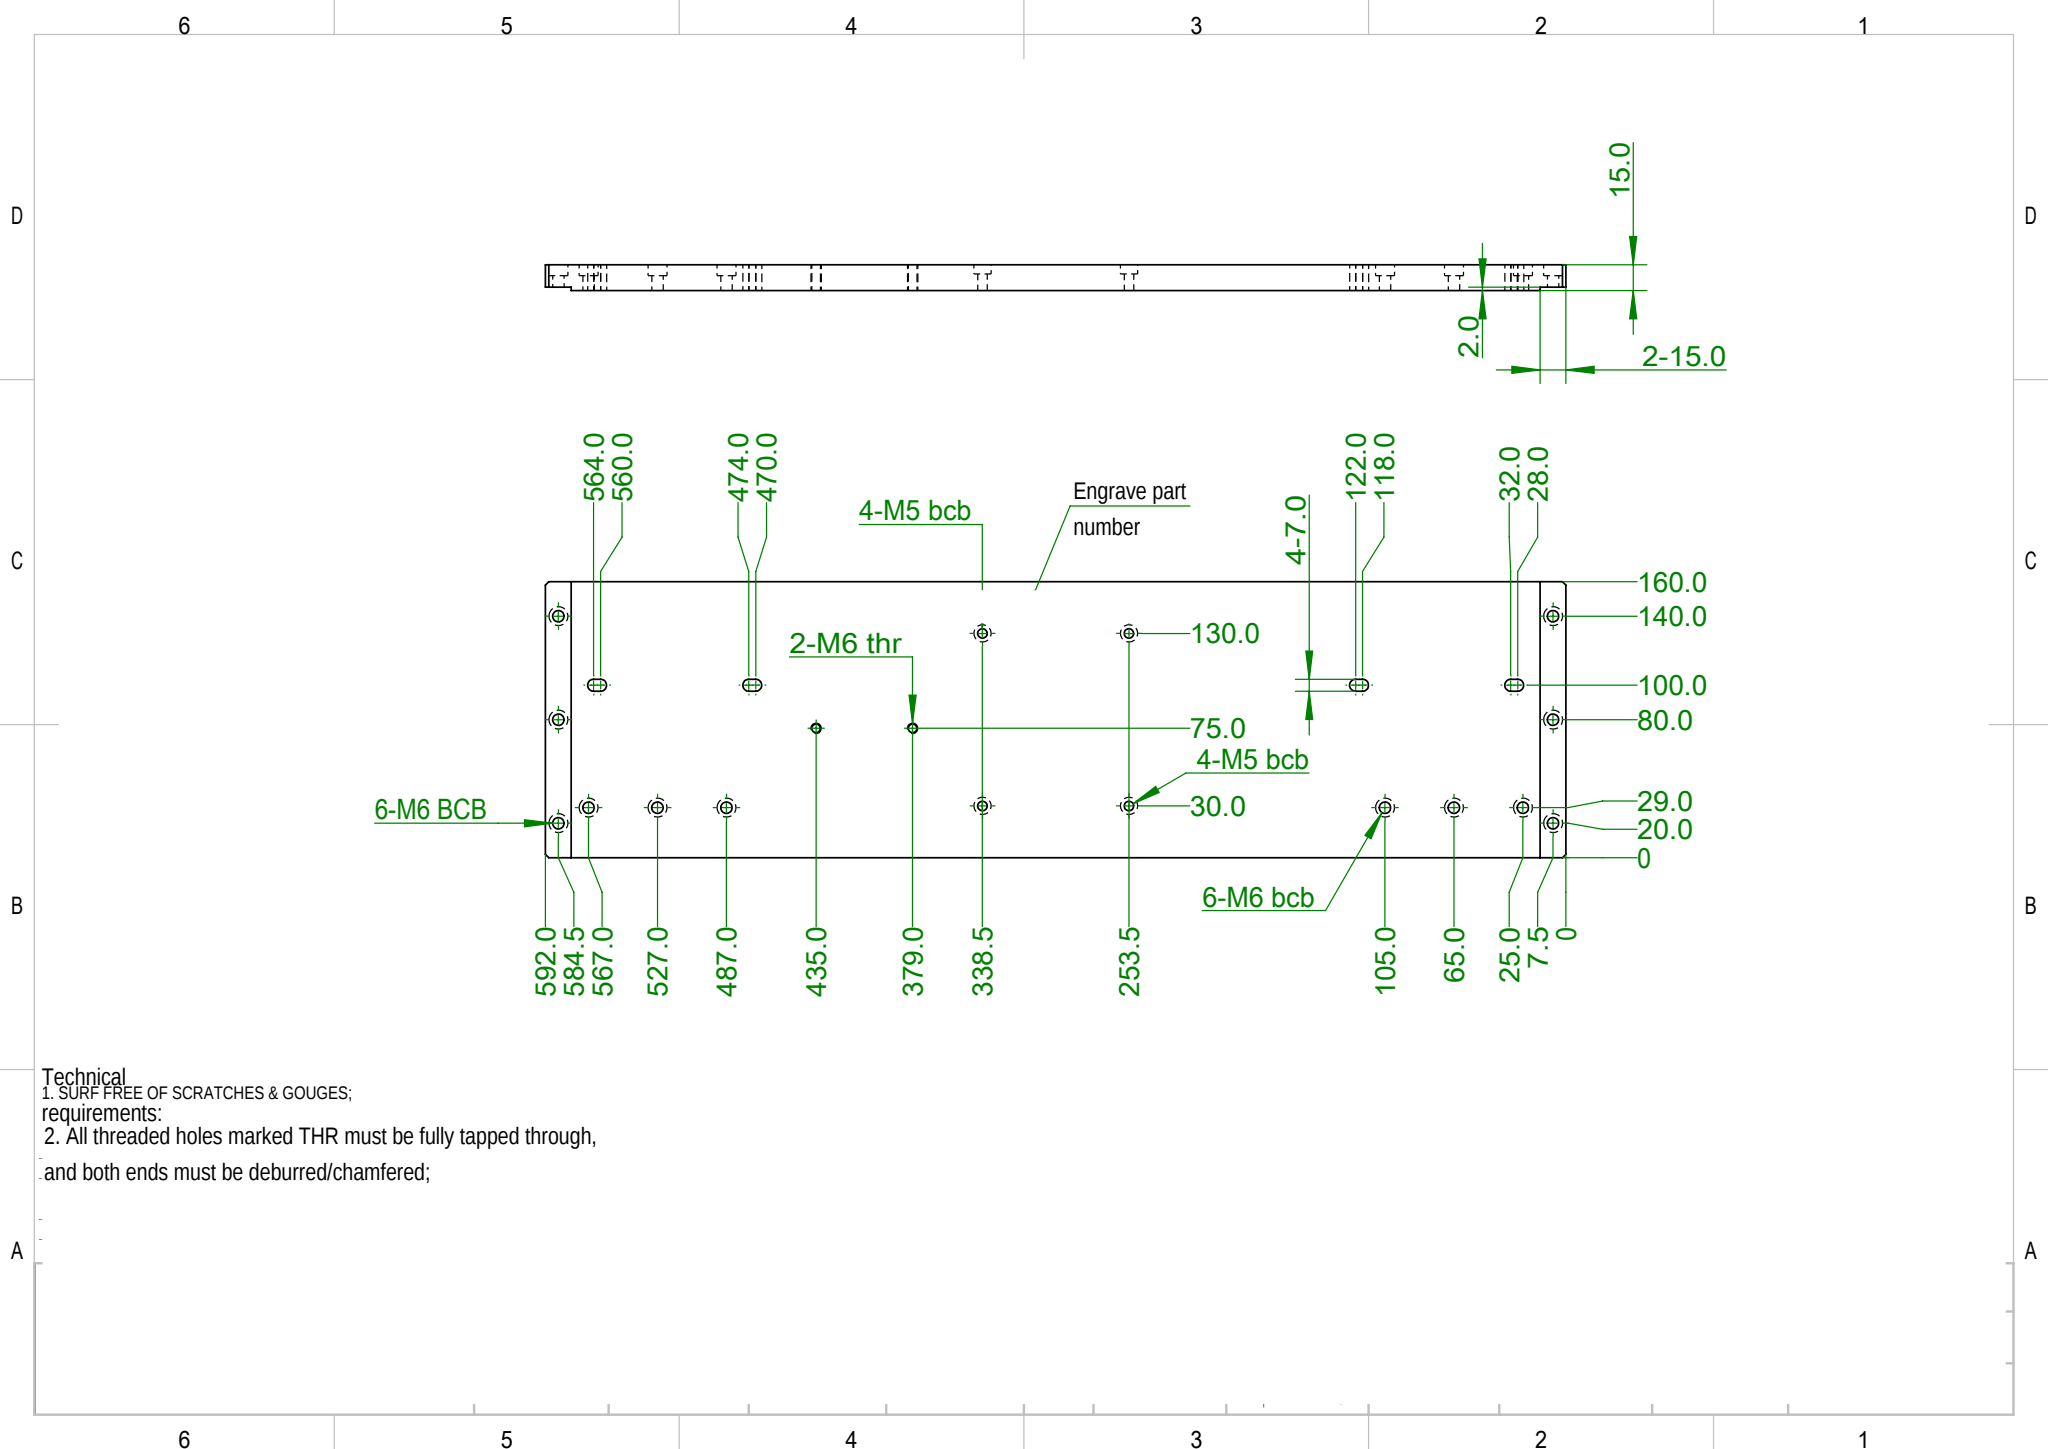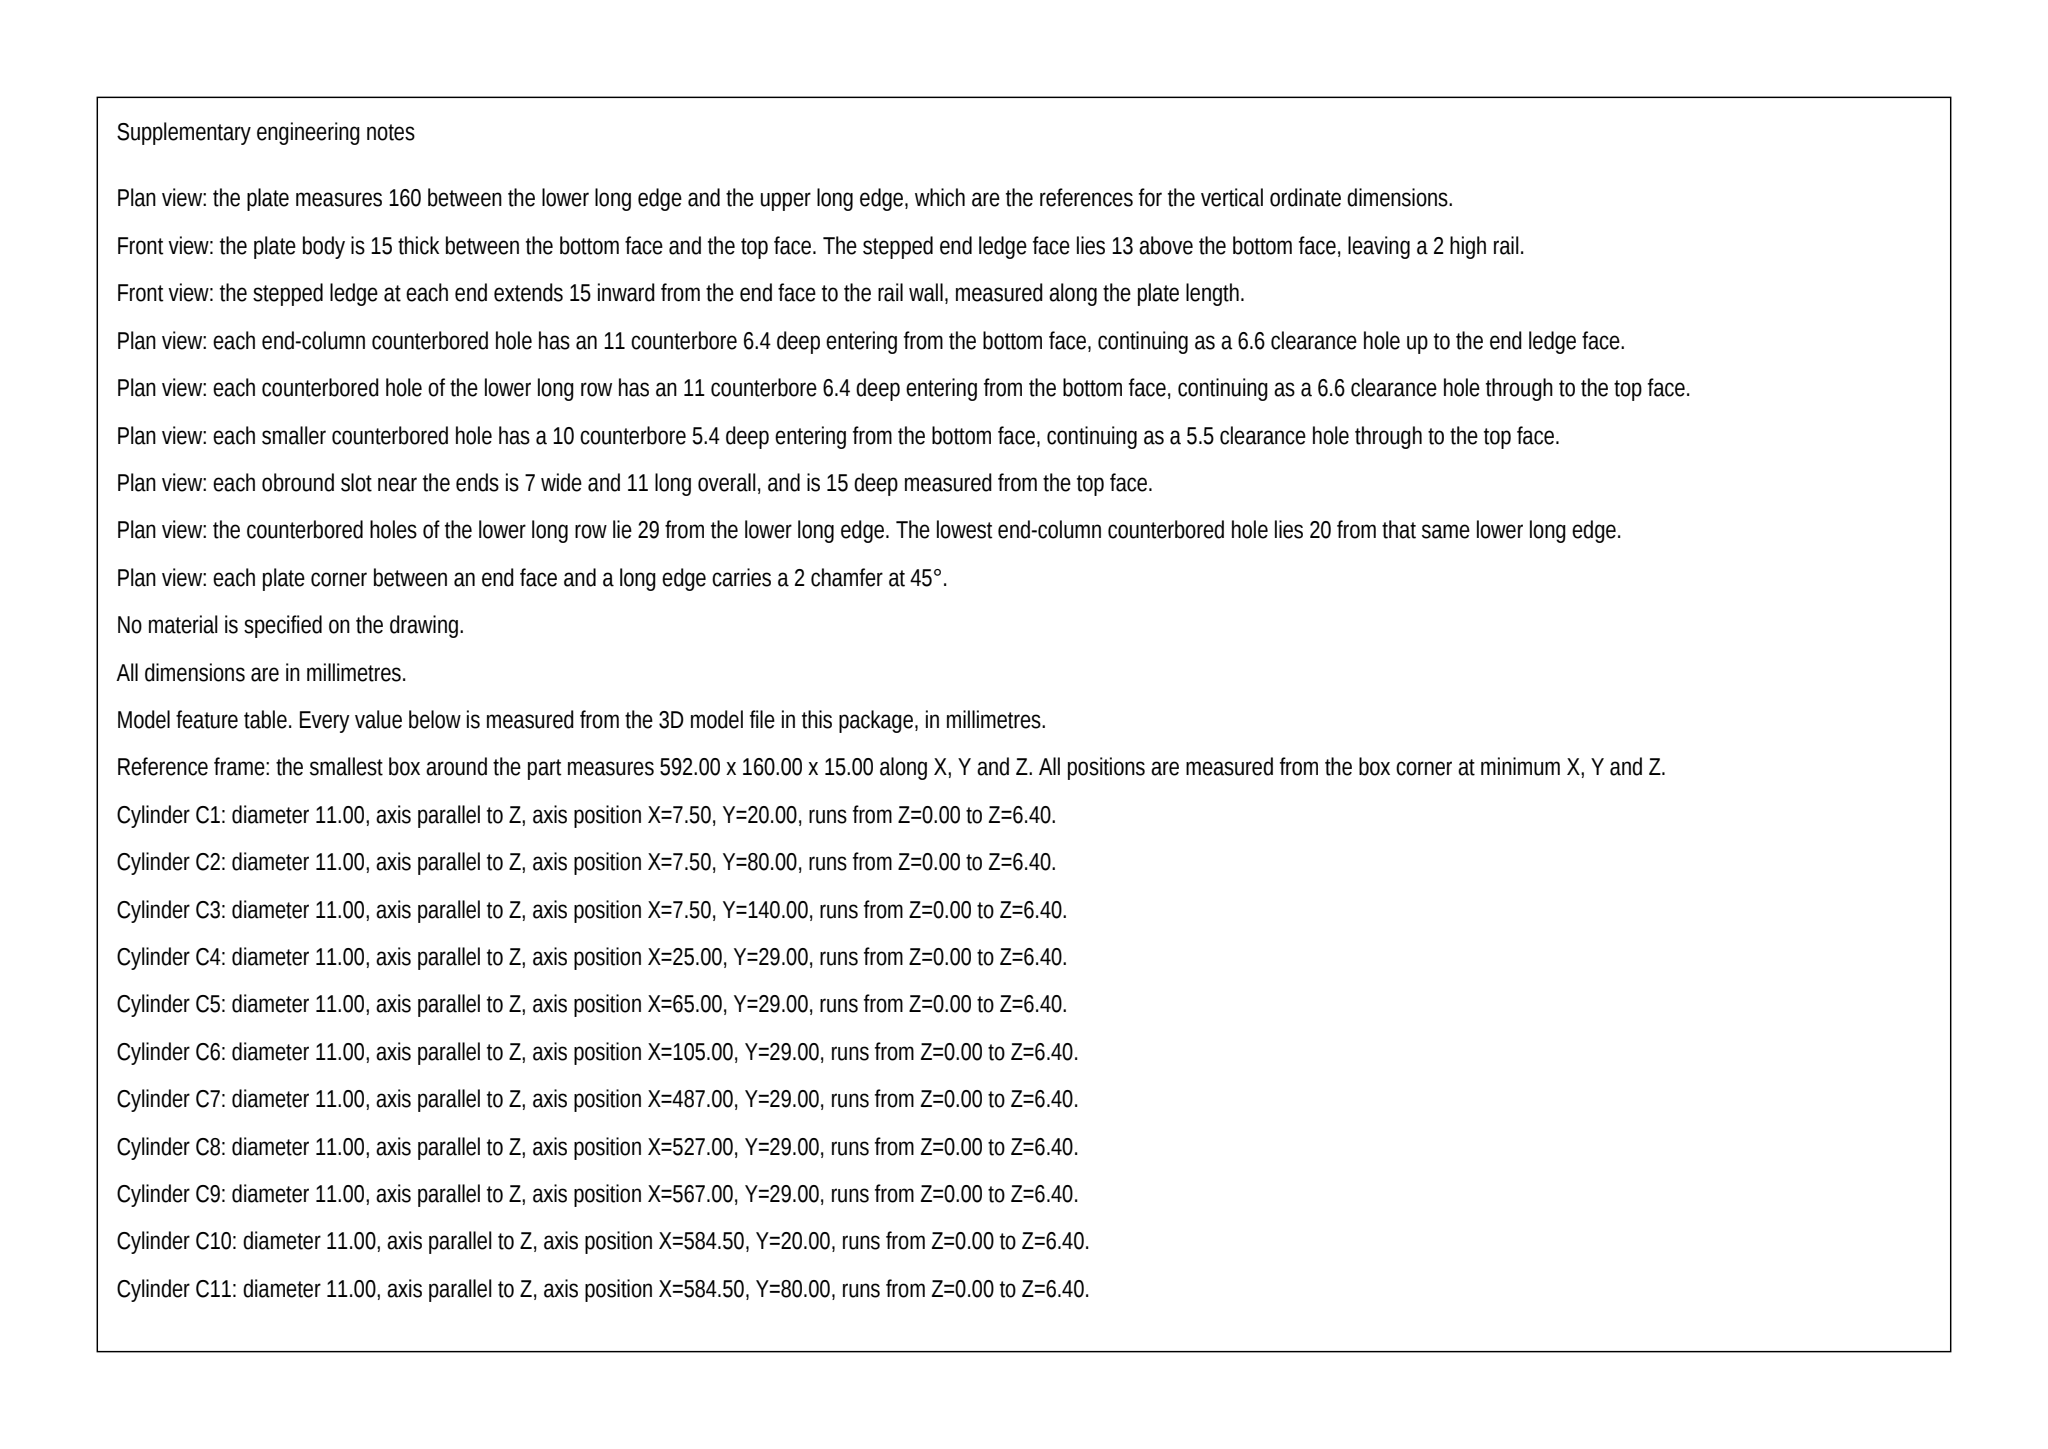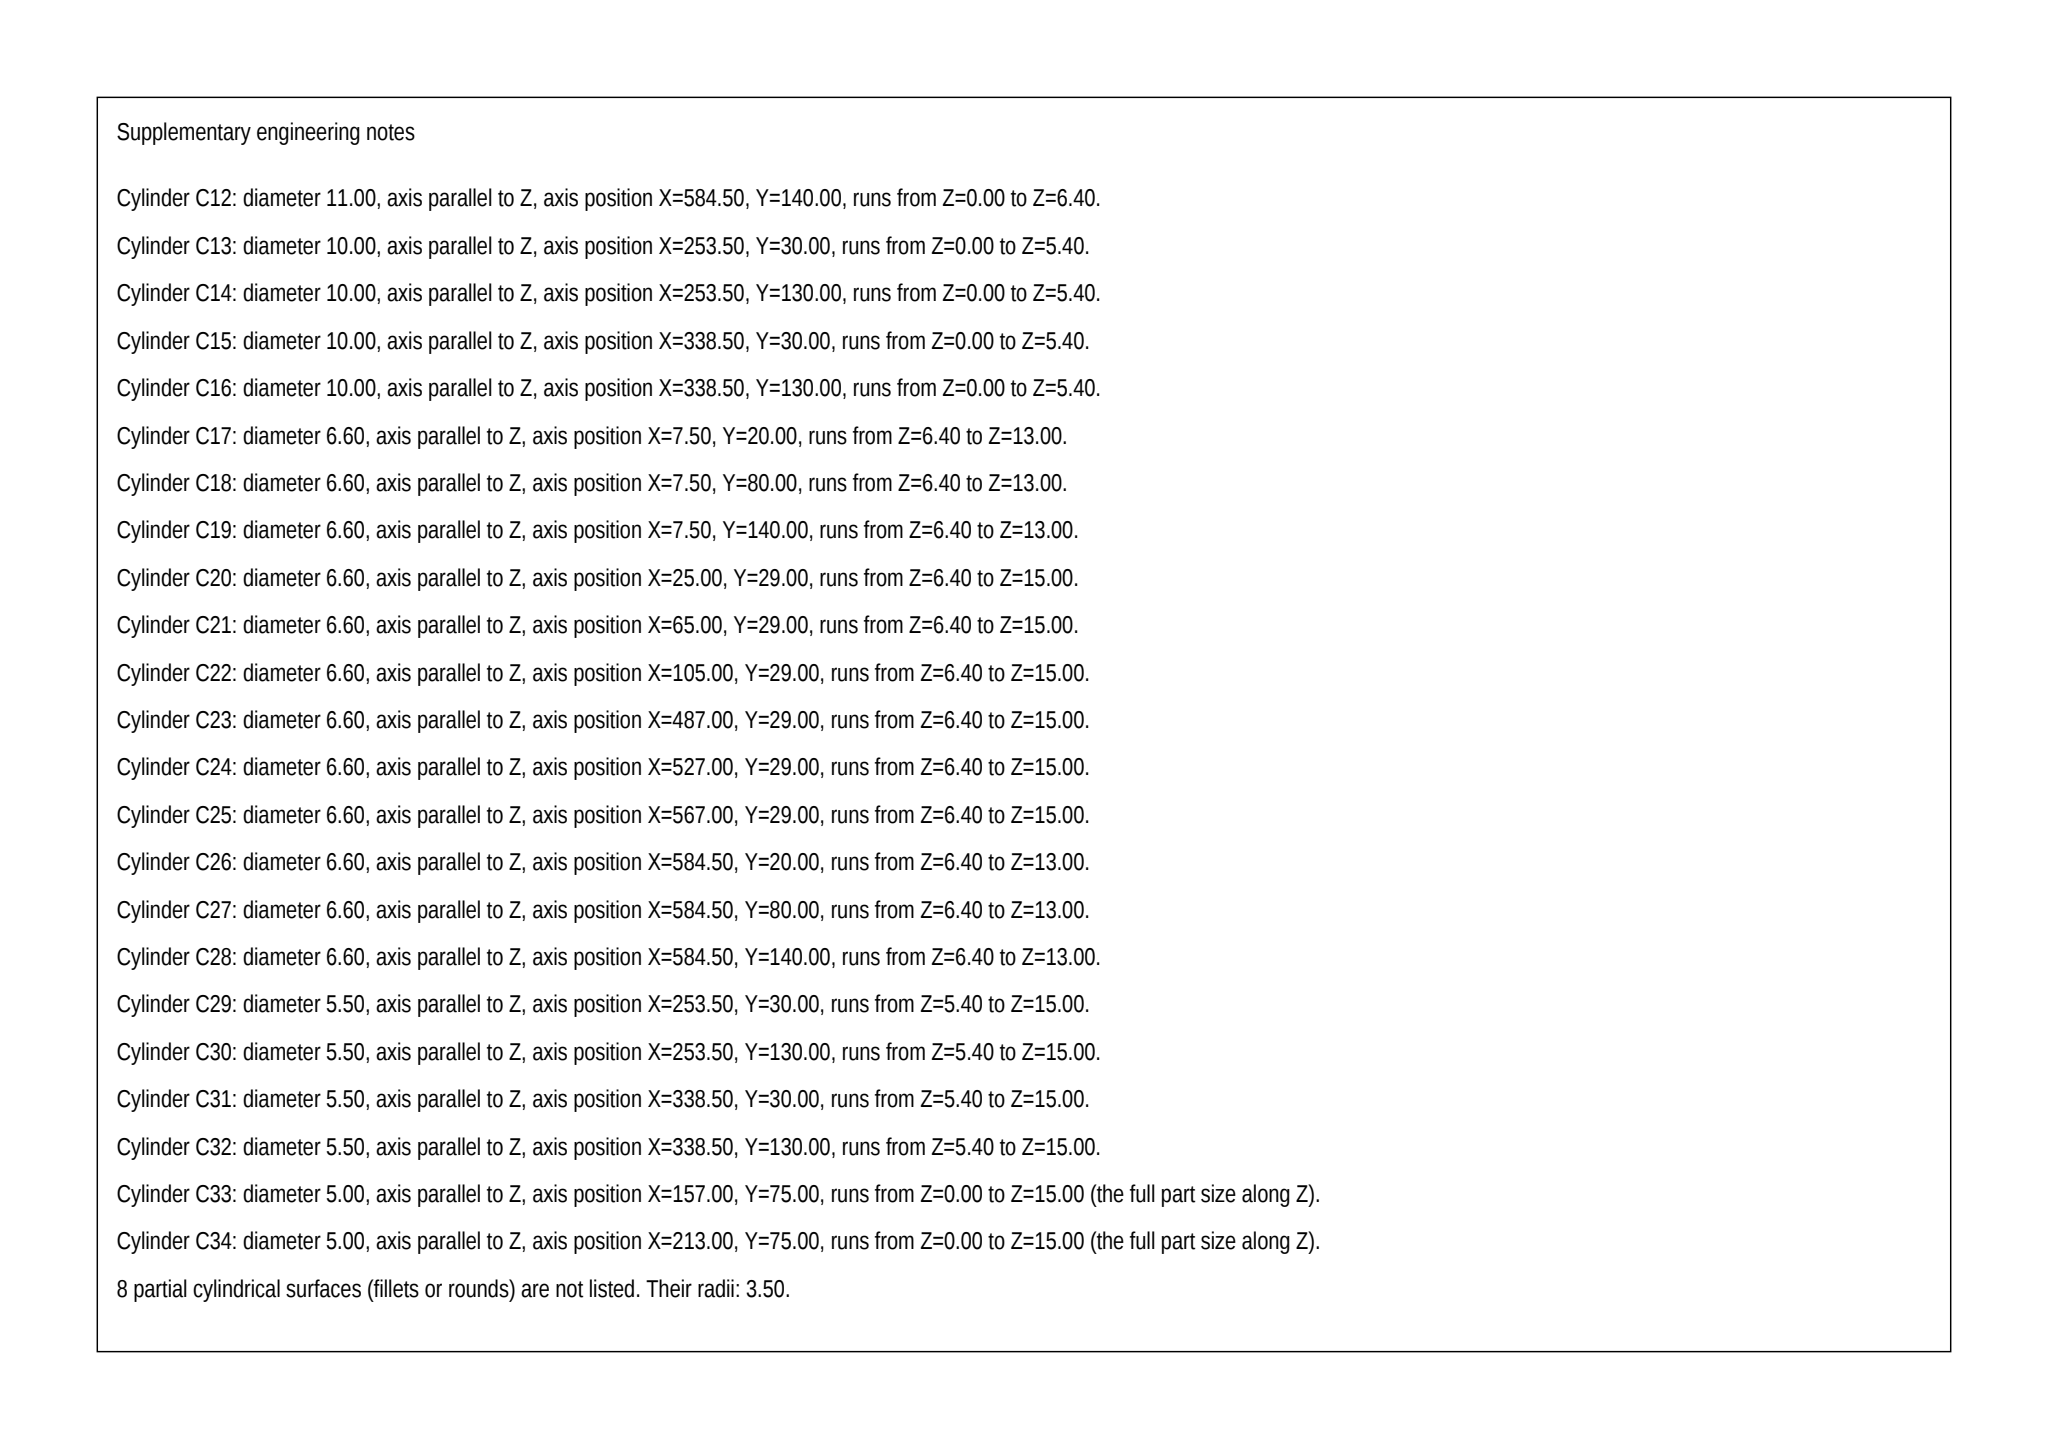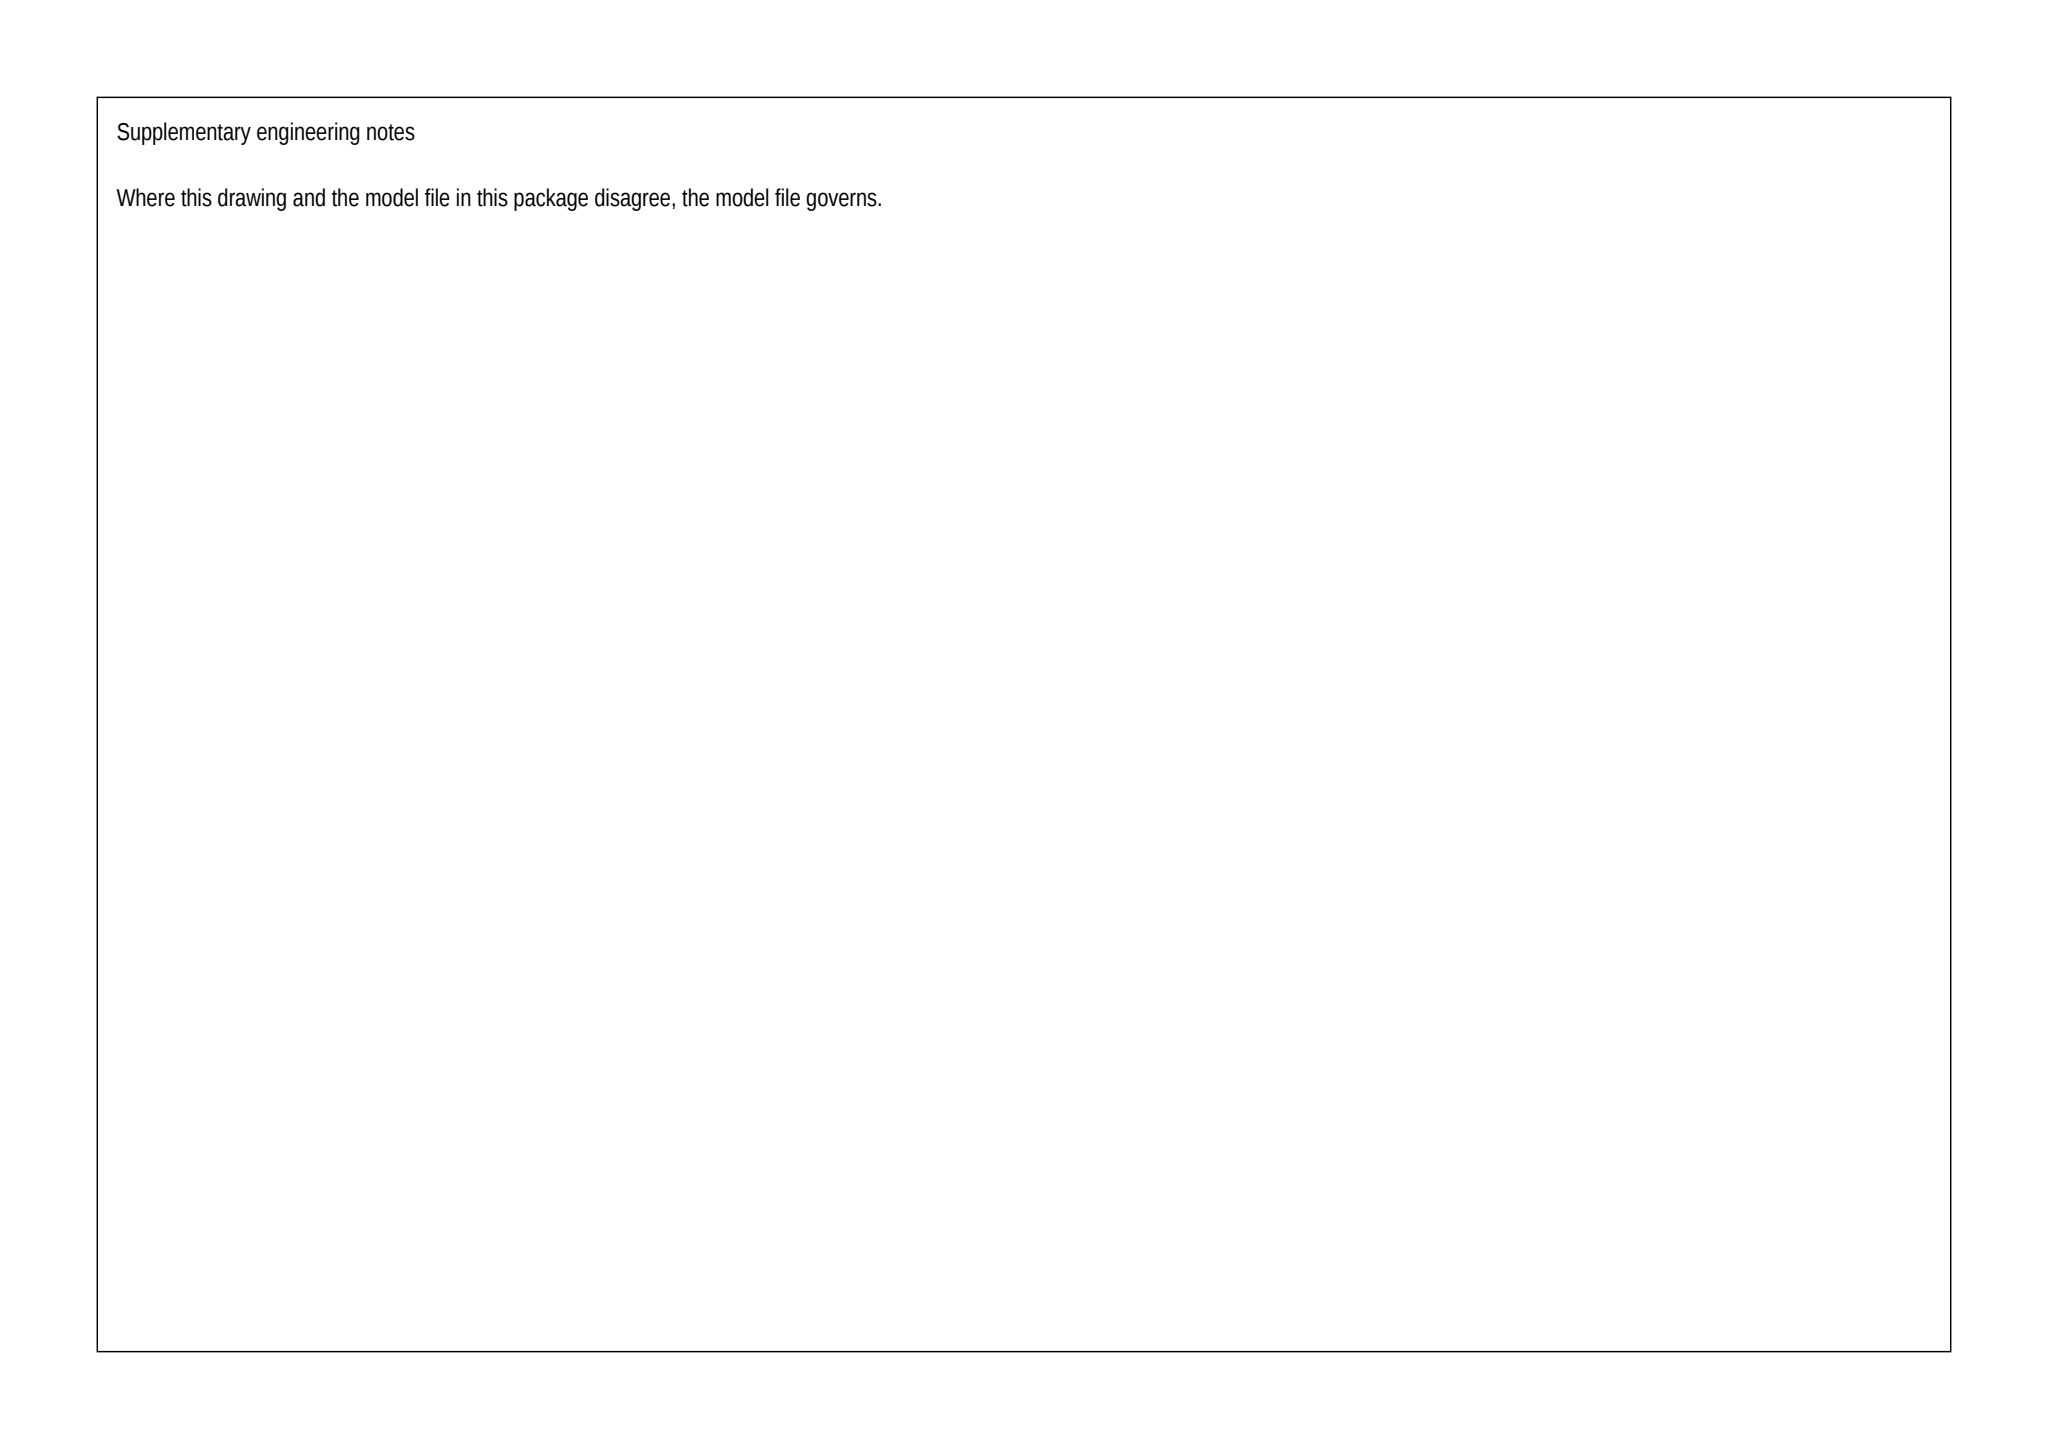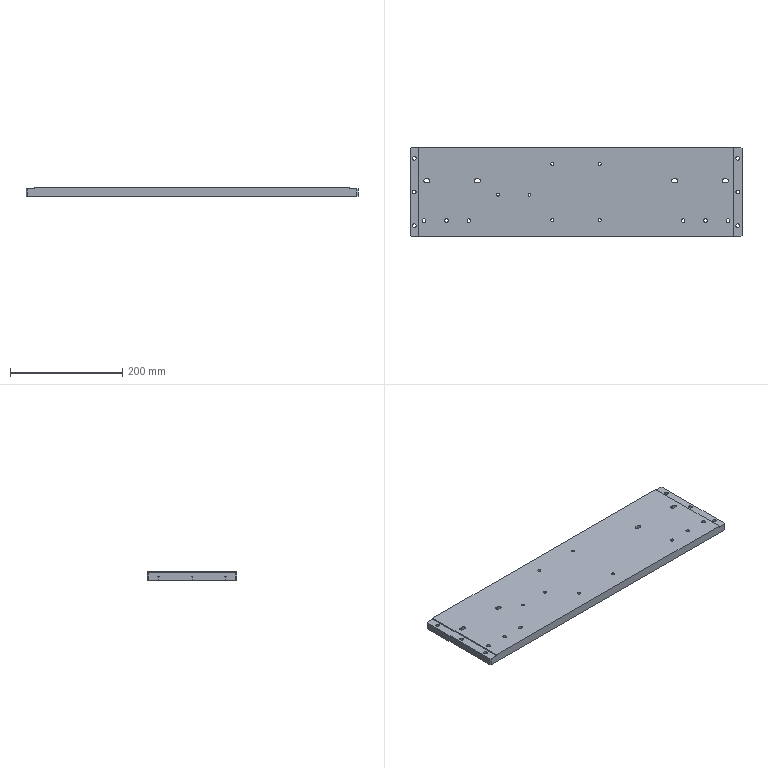Part | SolidWorks | mm | 1 solid | 118 faces | box 592 x 160 x 15 mm | volume 1393490 mm3 | cylinder 80 | plane 38 | commonest cylinder face diameters 11 x24 6.6 x24 7 x12 10 x8 5.5 x8 5 x4
Drawing notes:
12X Ø6.6 THRU, C'BORE Ø11.0 DEEP 6.4 from top face; located from bbox min corner at (X7.5,Y20), (X7.5,Y80), (X7.5,Y140), (X584.5,Y20), (X584.5,Y80), (X584.5,Y140), and (X25,Y29), (X65,Y29), (X105,Y29), (X487,Y29), (X527,Y29), (X567,Y29). | from the solid: cylinders dia 6.6 (12 locations, len 6.6/8.6) with coaxial dia 11.0 depth 6.4 at same XY
4X Ø5.5 THRU, C'BORE Ø10.0 DEEP 5.4 from top face; located from bbox min corner at (X253.5,Y30), (X253.5,Y130), (X338.5,Y30), (X338.5,Y130). | from the solid: cylinders dia 5.5 len 9.6 at (253.5/338.5, 30/130) with coaxial dia 10.0 depth 5.4
4X Ø7.0 THRU slots, full 15.0 plate thickness, slot centerline Y=100.0 from bbox min corner; end-radius centers at X=28.0 & 32.0, X=118.0 & 122.0, X=470.0 & 474.0, X=560.0 & 564.0. | from the solid: cylinders dia 7.0 axis z len 15.0 at y=100.0, x=28/32, 118/122, 470/474, 560/564
2X M6 TAPPED THRU (tap drill Ø5.0 through 15.0 thickness), located from bbox min corner at (X157.0,Y75.0) and (X213.0,Y75.0). | from the solid: cylinders dia 5.0 axis z len 15.0 at (157.0,75.0) and (213.0,75.0)
All dimensions are in millimetres; overall part size 592.0 x 160.0 x 15.0. | from the solid: bbox_xyz [592.0,160.0,15.0] with units mm
SLOT: 4X Ø7.0 THRU slots, full 15.0 plate thickness; slot centerline Y=100.0 from bbox min corner; end-radius centers at X=118.0 and X=122.0 from bbox min corner (X0,Y0 = bbox min corner). | from the solid: cylinders dia 7.0, axis z, pos (118.0,100.0) and (122.0,100.0), length 15.0 = full 15.0 plate thickness; bbox_xyz 592.0 x 160.0 x 15.0
build123d program:
from build123d import *

# Parameters (mm, degrees)
SKETCH1_W                                       = 590
SKETCH1_H                                       = 160
BOSS_EXTRUDE1_DEPTH                             = 15
SKETCH2_W                                       = 14
SKETCH2_H                                       = 160
CUT_EXTRUDE1_DEPTH                              = 2
M5_HEX_SOCKET_HEAD_CAP_SCREW_CBORE1_D           = 5.5
M5_HEX_SOCKET_HEAD_CAP_SCREW_CBORE1_CBORE_D     = 10
M5_HEX_SOCKET_HEAD_CAP_SCREW_CBORE1_CBORE_DEPTH = 5.4
MOVE_FACE1_BY                                   = 1
MOVE_FACE2_BY                                   = 1
CUT_EXTRUDE3_DEPTH                              = 111
M6_HEX_SOCKET_HEAD_CAP_SCREW_CBORE1_D           = 6.6
M6_HEX_SOCKET_HEAD_CAP_SCREW_CBORE1_CBORE_D     = 11
M6_HEX_SOCKET_HEAD_CAP_SCREW_CBORE1_CBORE_DEPTH = 6.4
M6_HEX_SOCKET_HEAD_CAP_SCREW_CBORE2_D           = 6.6
M6_HEX_SOCKET_HEAD_CAP_SCREW_CBORE2_CBORE_D     = 11
M6_HEX_SOCKET_HEAD_CAP_SCREW_CBORE2_CBORE_DEPTH = 6.4
M6_TAPPED_HOLE1_D                               = 5
CHAMFER1_SIZE                                   = 2


with BuildPart() as part:
    # Sketch1 → Boss-Extrude1 (new body)
    with BuildSketch(Plane.XY):
        Rectangle(SKETCH1_W, SKETCH1_H)
    extrude(amount=BOSS_EXTRUDE1_DEPTH)

    # Sketch2 → Cut-Extrude1 (cut)
    with BuildSketch(Plane.XY.offset(15)):
        with Locations((-288, 0)):
            Rectangle(SKETCH2_W, SKETCH2_H)
        with Locations((288, 0)):
            Rectangle(SKETCH2_W, SKETCH2_H)
    extrude(amount=-CUT_EXTRUDE1_DEPTH, mode=Mode.SUBTRACT)

    # M5 Hex Socket Head Cap Screw CBORE1 (through all)
    with Locations(Plane(origin=(42.5, 50, 0), x_dir=(-1, 0, 0), z_dir=(0, 0, -1))):
        with Locations((0, 0), (85, 0), (0, -100), (85, -100)):
            CounterBoreHole(M5_HEX_SOCKET_HEAD_CAP_SCREW_CBORE1_D / 2, M5_HEX_SOCKET_HEAD_CAP_SCREW_CBORE1_CBORE_D / 2, M5_HEX_SOCKET_HEAD_CAP_SCREW_CBORE1_CBORE_DEPTH)

    # Move Face1: a face moved outward by 1.0
    extrude(part.faces().sort_by_distance((-295, 0, 6.5))[0], amount=MOVE_FACE1_BY, dir=(-1, 0, 0))

    # Move Face2: a face moved outward by 1.0
    extrude(part.faces().sort_by_distance((295, 0, 6.5))[0], amount=MOVE_FACE2_BY, dir=(1, 0, 0))

    # Sketch10 → Cut-Extrude3 (cut)
    with BuildSketch(Plane.XY.offset(15)):
        with BuildLine():
            Line((-268, 23.5), (-264, 23.5))
            ThreePointArc((-264, 23.5), (-260.5, 20), (-264, 16.5))
            Line((-264, 16.5), (-268, 16.5))
            ThreePointArc((-268, 16.5), (-271.5, 20), (-268, 23.5))
        make_face()
        with BuildLine():
            Line((-178, 23.5), (-174, 23.5))
            ThreePointArc((-174, 23.5), (-170.5, 20), (-174, 16.5))
            Line((-174, 16.5), (-178, 16.5))
            ThreePointArc((-178, 16.5), (-181.5, 20), (-178, 23.5))
        make_face()
    cut_extrude3 = extrude(amount=-CUT_EXTRUDE3_DEPTH, mode=Mode.SUBTRACT)

    # Mirror1: Cut-Extrude3 across plane
    add(cut_extrude3.mirror(Plane(origin=(0, 0, 0), x_dir=(0, 0, 1), z_dir=(1, 0, 0))), mode=Mode.SUBTRACT)

    # M6 Hex Socket Head Cap Screw CBORE1 (through all)
    with Locations(Plane(origin=(0, 0, 0), x_dir=(-1, 0, 0), z_dir=(0, 0, -1))):
        with Locations((271, -51), (231, -51), (191, -51), (-191, -51), (-231, -51), (-271, -51)):
            CounterBoreHole(M6_HEX_SOCKET_HEAD_CAP_SCREW_CBORE1_D / 2, M6_HEX_SOCKET_HEAD_CAP_SCREW_CBORE1_CBORE_D / 2, M6_HEX_SOCKET_HEAD_CAP_SCREW_CBORE1_CBORE_DEPTH)

    # M6 Hex Socket Head Cap Screw CBORE2 (through all)
    with Locations(Plane(origin=(0, 0, 0), x_dir=(-1, 0, 0), z_dir=(0, 0, -1))):
        with Locations((288.5, 60), (288.5, 0), (288.5, -60), (-288.5, 60), (-288.5, 0), (-288.5, -60)):
            CounterBoreHole(M6_HEX_SOCKET_HEAD_CAP_SCREW_CBORE2_D / 2, M6_HEX_SOCKET_HEAD_CAP_SCREW_CBORE2_CBORE_D / 2, M6_HEX_SOCKET_HEAD_CAP_SCREW_CBORE2_CBORE_DEPTH)

    # M6 Tapped Hole1 (through all)
    with Locations(Plane.XY.offset(15)):
        with Locations((-83, -5), (-139, -5)):
            Hole(M6_TAPPED_HOLE1_D / 2)

    # Chamfer1
    chamfer1_edges = [part.edges().sort_by_distance(p)[0] for p in [
        (-296, -80, 6.5),
        (-296, 80, 6.5),
        (296, -80, 6.5),
        (296, 80, 6.5),
    ]]
    chamfer(chamfer1_edges, length=CHAMFER1_SIZE)


solid = part.part